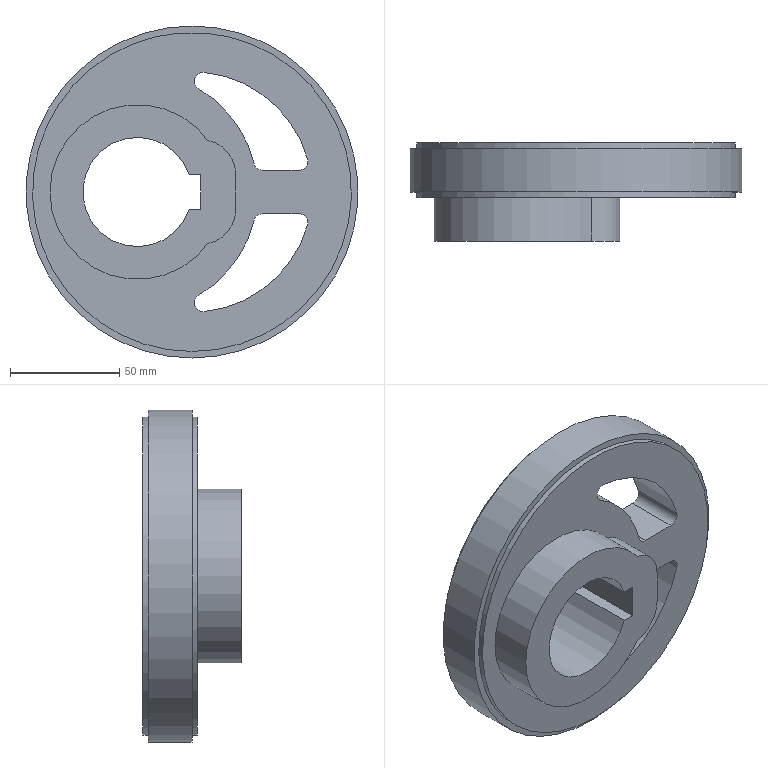Component | NX | SHEAVE | 1 solid | 28 faces | volume 407857 mm3 | cylinder 17 | plane 11 | commonest cylinder face diameters 8 x6 110 x4 146 x2 32 x2 152 x1 80 x1 50 x1